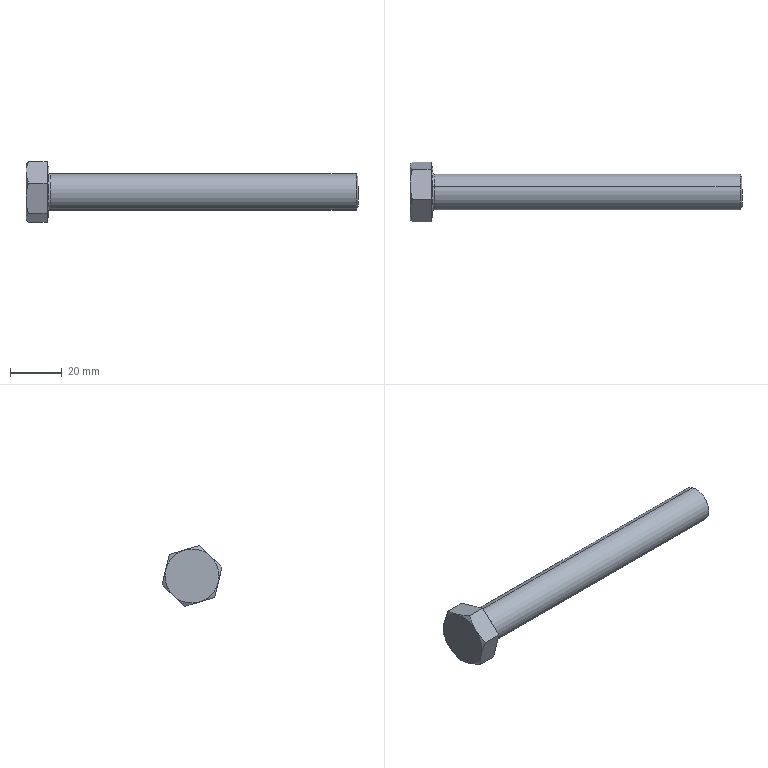Component | SolidWorks | GB_T5785-2016[HexHeadBoltFineThread(M14_1.5)_120]-1 | 1 solid | 24 faces | box 128.8 x 23.23 x 23.59 mm | volume 21766 mm3 | cone 10 | plane 10 | torus 2 | cylinder 2 | commonest cylinder face diameters 14 x2
STEP:
#1=COLOUR_RGB('',0.7922,0.8196,0.9333);
#2=FILL_AREA_STYLE_COLOUR('',#1);
#3=FILL_AREA_STYLE('',(#2));
#4=SURFACE_STYLE_FILL_AREA(#3);
#5=SURFACE_SIDE_STYLE('',(#4));
#6=SURFACE_STYLE_USAGE(.BOTH.,#5);
#7=PRESENTATION_STYLE_ASSIGNMENT((#6));
#8=CARTESIAN_POINT('',(18.543,31.116,10.34));
#9=VERTEX_POINT('',#8);
#10=CARTESIAN_POINT('',(18.543,30.987,9.91));
#11=VERTEX_POINT('',#10);
#12=CARTESIAN_POINT('',(18.543,31.052,10.125));
#13=DIRECTION('',(-1.,-0.,-0.));
#14=DIRECTION('',(-0.,0.2864,0.9581));
#15=AXIS2_PLACEMENT_3D('',#12,#13,#14);
#16=CIRCLE('',#15,0.2244);
#17=EDGE_CURVE('',#9,#11,#16,.T.);
#18=ORIENTED_EDGE('',*,*,#17,.T.);
#19=CARTESIAN_POINT('',(18.513,30.973,9.861));
#20=VERTEX_POINT('',#19);
#21=CARTESIAN_POINT('',(18.513,30.973,9.861));
#22=DIRECTION('',(-0.5,-0.2481,-0.8297));
#23=VECTOR('',#22,39.37);
#24=LINE('',#21,#23);
#25=EDGE_CURVE('',#11,#20,#24,.T.);
#26=ORIENTED_EDGE('',*,*,#25,.T.);
#27=CARTESIAN_POINT('',(18.513,31.13,10.389));
#28=VERTEX_POINT('',#27);
#29=CARTESIAN_POINT('',(18.513,31.052,10.125));
#30=DIRECTION('',(-1.,-0.,-0.));
#31=DIRECTION('',(-0.,0.2864,0.9581));
#32=AXIS2_PLACEMENT_3D('',#29,#30,#31);
#33=CIRCLE('',#32,0.2756);
#34=EDGE_CURVE('',#28,#20,#33,.T.);
#35=ORIENTED_EDGE('',*,*,#34,.F.);
#36=CARTESIAN_POINT('',(18.513,31.13,10.389));
#37=DIRECTION('',(-0.5,0.2481,0.8297));
#38=VECTOR('',#37,39.37);
#39=LINE('',#36,#38);
#40=EDGE_CURVE('',#9,#28,#39,.T.);
#41=ORIENTED_EDGE('',*,*,#40,.F.);
#42=EDGE_LOOP('',(#18,#26,#35,#41));
#43=FACE_OUTER_BOUND('',#42,.T.);
#44=CARTESIAN_POINT('',(18.513,31.052,10.125));
#45=DIRECTION('',(-1.,-0.,-0.));
#46=DIRECTION('',(-0.,0.2864,0.9581));
#47=AXIS2_PLACEMENT_3D('',#44,#45,#46);
#48=CONICAL_SURFACE('',#47,0.2756,1.047);
#49=ADVANCED_FACE('',(#43),#48,.T.);
#50=CARTESIAN_POINT('',(13.842,31.13,10.389));
#51=VERTEX_POINT('',#50);
#52=CARTESIAN_POINT('',(13.842,30.973,9.861));
#53=VERTEX_POINT('',#52);
#54=CARTESIAN_POINT('',(13.842,31.052,10.125));
#55=DIRECTION('',(1.,0.,0.));
#56=DIRECTION('',(0.,-0.2864,-0.9581));
#57=AXIS2_PLACEMENT_3D('',#54,#55,#56);
#58=CIRCLE('',#57,0.2756);
#59=EDGE_CURVE('',#51,#53,#58,.T.);
#60=ORIENTED_EDGE('',*,*,#59,.F.);
#61=CARTESIAN_POINT('',(13.818,31.137,10.412));
#62=VERTEX_POINT('',#61);
#63=CARTESIAN_POINT('',(13.842,31.137,10.412));
#64=DIRECTION('',(-0.,0.9581,-0.2864));
#65=DIRECTION('',(0.,0.2864,0.9581));
#66=AXIS2_PLACEMENT_3D('',#63,#64,#65);
#67=CIRCLE('',#66,0.02362);
#68=EDGE_CURVE('',#51,#62,#67,.T.);
#69=ORIENTED_EDGE('',*,*,#68,.T.);
#70=CARTESIAN_POINT('',(13.818,30.966,9.839));
#71=VERTEX_POINT('',#70);
#72=CARTESIAN_POINT('',(13.818,31.052,10.125));
#73=DIRECTION('',(-1.,-0.,-0.));
#74=DIRECTION('',(0.,-0.2864,-0.9581));
#75=AXIS2_PLACEMENT_3D('',#72,#73,#74);
#76=CIRCLE('',#75,0.2992);
#77=EDGE_CURVE('',#71,#62,#76,.T.);
#78=ORIENTED_EDGE('',*,*,#77,.F.);
#79=CARTESIAN_POINT('',(13.842,30.966,9.839));
#80=DIRECTION('',(0.,-0.9581,0.2864));
#81=DIRECTION('',(0.,-0.2864,-0.9581));
#82=AXIS2_PLACEMENT_3D('',#79,#80,#81);
#83=CIRCLE('',#82,0.02362);
#84=EDGE_CURVE('',#53,#71,#83,.T.);
#85=ORIENTED_EDGE('',*,*,#84,.F.);
#86=EDGE_LOOP('',(#60,#69,#78,#85));
#87=FACE_OUTER_BOUND('',#86,.T.);
#88=CARTESIAN_POINT('',(13.842,31.052,10.125));
#89=DIRECTION('',(1.,0.,0.));
#90=DIRECTION('',(0.,-0.2864,-0.9581));
#91=AXIS2_PLACEMENT_3D('',#88,#89,#90);
#92=TOROIDAL_SURFACE('',#91,0.2992,0.02362);
#93=ADVANCED_FACE('',(#87),#92,.F.);
#94=CARTESIAN_POINT('',(13.818,31.162,10.496));
#95=VERTEX_POINT('',#94);
#96=CARTESIAN_POINT('',(13.818,30.941,9.755));
#97=VERTEX_POINT('',#96);
#98=CARTESIAN_POINT('',(13.818,31.052,10.125));
#99=DIRECTION('',(-1.,-0.,-0.));
#100=DIRECTION('',(-0.,0.2864,0.9581));
#101=AXIS2_PLACEMENT_3D('',#98,#99,#100);
#102=CIRCLE('',#101,0.3866);
#103=EDGE_CURVE('',#95,#97,#102,.T.);
#104=ORIENTED_EDGE('',*,*,#103,.T.);
#105=CARTESIAN_POINT('',(13.795,30.937,9.742));
#106=VERTEX_POINT('',#105);
#107=CARTESIAN_POINT('',(13.795,30.937,9.742));
#108=DIRECTION('',(-0.866,-0.1432,-0.4791));
#109=VECTOR('',#108,39.37);
#110=LINE('',#107,#109);
#111=EDGE_CURVE('',#97,#106,#110,.T.);
#112=ORIENTED_EDGE('',*,*,#111,.T.);
#113=CARTESIAN_POINT('',(13.795,31.166,10.509));
#114=VERTEX_POINT('',#113);
#115=CARTESIAN_POINT('',(13.795,31.052,10.125));
#116=DIRECTION('',(-1.,-0.,-0.));
#117=DIRECTION('',(-0.,0.2864,0.9581));
#118=AXIS2_PLACEMENT_3D('',#115,#116,#117);
#119=CIRCLE('',#118,0.4003);
#120=EDGE_CURVE('',#114,#106,#119,.T.);
#121=ORIENTED_EDGE('',*,*,#120,.F.);
#122=CARTESIAN_POINT('',(13.795,31.166,10.509));
#123=DIRECTION('',(-0.866,0.1432,0.4791));
#124=VECTOR('',#123,39.37);
#125=LINE('',#122,#124);
#126=EDGE_CURVE('',#95,#114,#125,.T.);
#127=ORIENTED_EDGE('',*,*,#126,.F.);
#128=EDGE_LOOP('',(#104,#112,#121,#127));
#129=FACE_OUTER_BOUND('',#128,.T.);
#130=CARTESIAN_POINT('',(13.795,31.052,10.125));
#131=DIRECTION('',(-1.,-0.,-0.));
#132=DIRECTION('',(-0.,0.2864,0.9581));
#133=AXIS2_PLACEMENT_3D('',#130,#131,#132);
#134=CONICAL_SURFACE('',#133,0.4003,0.5236);
#135=ADVANCED_FACE('',(#129),#134,.T.);
#136=ORIENTED_EDGE('',*,*,#34,.T.);
#137=CARTESIAN_POINT('',(13.472,30.973,9.861));
#138=DIRECTION('',(-1.,-0.,-0.));
#139=VECTOR('',#138,39.37);
#140=LINE('',#137,#139);
#141=EDGE_CURVE('',#20,#53,#140,.T.);
#142=ORIENTED_EDGE('',*,*,#141,.T.);
#143=CARTESIAN_POINT('',(13.842,31.052,10.125));
#144=DIRECTION('',(1.,0.,0.));
#145=DIRECTION('',(0.,-0.2864,-0.9581));
#146=AXIS2_PLACEMENT_3D('',#143,#144,#145);
#147=CIRCLE('',#146,0.2756);
#148=EDGE_CURVE('',#53,#51,#147,.T.);
#149=ORIENTED_EDGE('',*,*,#148,.T.);
#150=CARTESIAN_POINT('',(13.472,31.13,10.389));
#151=DIRECTION('',(-1.,-0.,-0.));
#152=VECTOR('',#151,39.37);
#153=LINE('',#150,#152);
#154=EDGE_CURVE('',#28,#51,#153,.T.);
#155=ORIENTED_EDGE('',*,*,#154,.F.);
#156=EDGE_LOOP('',(#136,#142,#149,#155));
#157=FACE_OUTER_BOUND('',#156,.T.);
#158=CARTESIAN_POINT('',(13.472,31.052,10.125));
#159=DIRECTION('',(-1.,-0.,-0.));
#160=DIRECTION('',(-0.,0.2864,0.9581));
#161=AXIS2_PLACEMENT_3D('',#158,#159,#160);
#162=CYLINDRICAL_SURFACE('',#161,0.2756);
#163=ADVANCED_FACE('',(#157),#162,.T.);
#164=ORIENTED_EDGE('',*,*,#141,.F.);
#165=CARTESIAN_POINT('',(18.513,31.052,10.125));
#166=DIRECTION('',(-1.,-0.,-0.));
#167=DIRECTION('',(-0.,0.2864,0.9581));
#168=AXIS2_PLACEMENT_3D('',#165,#166,#167);
#169=CIRCLE('',#168,0.2756);
#170=EDGE_CURVE('',#20,#28,#169,.T.);
#171=ORIENTED_EDGE('',*,*,#170,.T.);
#172=ORIENTED_EDGE('',*,*,#154,.T.);
#173=ORIENTED_EDGE('',*,*,#59,.T.);
#174=EDGE_LOOP('',(#164,#171,#172,#173));
#175=FACE_OUTER_BOUND('',#174,.T.);
#176=CARTESIAN_POINT('',(13.472,31.052,10.125));
#177=DIRECTION('',(-1.,-0.,-0.));
#178=DIRECTION('',(-0.,0.2864,0.9581));
#179=AXIS2_PLACEMENT_3D('',#176,#177,#178);
#180=CYLINDRICAL_SURFACE('',#179,0.2756);
#181=ADVANCED_FACE('',(#175),#180,.T.);
#182=CARTESIAN_POINT('',(13.795,31.162,9.661));
#183=VERTEX_POINT('',#182);
#184=CARTESIAN_POINT('',(13.795,31.509,9.988));
#185=VERTEX_POINT('',#184);
#186=CARTESIAN_POINT('',(13.795,31.162,9.661));
#187=DIRECTION('',(-0.,0.7271,0.6865));
#188=VECTOR('',#187,39.37);
#189=LINE('',#186,#188);
#190=EDGE_CURVE('',#183,#185,#189,.T.);
#191=ORIENTED_EDGE('',*,*,#190,.F.);
#192=CARTESIAN_POINT('',(13.509,31.162,9.661));
#193=VERTEX_POINT('',#192);
#194=CARTESIAN_POINT('',(13.818,31.162,9.661));
#195=DIRECTION('',(-1.,-0.,-0.));
#196=VECTOR('',#195,39.37);
#197=LINE('',#194,#196);
#198=EDGE_CURVE('',#183,#193,#197,.T.);
#199=ORIENTED_EDGE('',*,*,#198,.T.);
#200=CARTESIAN_POINT('',(13.472,31.335,9.825));
#201=VERTEX_POINT('',#200);
#202=CARTESIAN_POINT('',(13.472,31.335,9.825));
#203=CARTESIAN_POINT('',(13.472,31.321,9.811));
#204=CARTESIAN_POINT('',(13.473,31.306,9.797));
#205=CARTESIAN_POINT('',(13.476,31.277,9.769));
#206=CARTESIAN_POINT('',(13.478,31.262,9.755));
#207=CARTESIAN_POINT('',(13.488,31.219,9.714));
#208=CARTESIAN_POINT('',(13.497,31.19,9.687));
#209=CARTESIAN_POINT('',(13.509,31.162,9.661));
#210=B_SPLINE_CURVE_WITH_KNOTS('',3,(#202,#203,#204,#205,#206,#207,#208,#209),.UNSPECIFIED.,.F.,.F.,(4,2,2,4),(0.006134,0.007662,0.00919,0.01225),.UNSPECIFIED.);
#211=EDGE_CURVE('',#201,#193,#210,.T.);
#212=ORIENTED_EDGE('',*,*,#211,.F.);
#213=CARTESIAN_POINT('',(13.509,31.509,9.988));
#214=VERTEX_POINT('',#213);
#215=CARTESIAN_POINT('',(13.509,31.509,9.988));
#216=CARTESIAN_POINT('',(13.497,31.481,9.962));
#217=CARTESIAN_POINT('',(13.488,31.452,9.935));
#218=CARTESIAN_POINT('',(13.475,31.394,9.88));
#219=CARTESIAN_POINT('',(13.472,31.365,9.853));
#220=CARTESIAN_POINT('',(13.472,31.335,9.825));
#221=B_SPLINE_CURVE_WITH_KNOTS('',3,(#215,#216,#217,#218,#219,#220),.UNSPECIFIED.,.F.,.F.,(4,2,4),(0.00000024,0.003067,0.006134),.UNSPECIFIED.);
#222=EDGE_CURVE('',#214,#201,#221,.T.);
#223=ORIENTED_EDGE('',*,*,#222,.F.);
#224=CARTESIAN_POINT('',(13.818,31.509,9.988));
#225=DIRECTION('',(-1.,-0.,-0.));
#226=VECTOR('',#225,39.37);
#227=LINE('',#224,#226);
#228=EDGE_CURVE('',#185,#214,#227,.T.);
#229=ORIENTED_EDGE('',*,*,#228,.F.);
#230=EDGE_LOOP('',(#191,#199,#212,#223,#229));
#231=FACE_OUTER_BOUND('',#230,.T.);
#232=CARTESIAN_POINT('',(13.818,31.162,9.661));
#233=DIRECTION('',(0.,-0.6865,0.7271));
#234=DIRECTION('',(0.,-0.7271,-0.6865));
#235=AXIS2_PLACEMENT_3D('',#232,#233,#234);
#236=PLANE('',#235);
#237=ADVANCED_FACE('',(#231),#236,.F.);
#238=CARTESIAN_POINT('',(13.795,31.399,10.453));
#239=VERTEX_POINT('',#238);
#240=CARTESIAN_POINT('',(13.795,31.509,9.988));
#241=DIRECTION('',(-0.,-0.231,0.973));
#242=VECTOR('',#241,39.37);
#243=LINE('',#240,#242);
#244=EDGE_CURVE('',#185,#239,#243,.T.);
#245=ORIENTED_EDGE('',*,*,#244,.F.);
#246=ORIENTED_EDGE('',*,*,#228,.T.);
#247=CARTESIAN_POINT('',(13.472,31.454,10.221));
#248=VERTEX_POINT('',#247);
#249=CARTESIAN_POINT('',(13.472,31.454,10.221));
#250=CARTESIAN_POINT('',(13.472,31.458,10.201));
#251=CARTESIAN_POINT('',(13.473,31.463,10.181));
#252=CARTESIAN_POINT('',(13.476,31.472,10.142));
#253=CARTESIAN_POINT('',(13.478,31.477,10.123));
#254=CARTESIAN_POINT('',(13.488,31.491,10.065));
#255=CARTESIAN_POINT('',(13.497,31.5,10.026));
#256=CARTESIAN_POINT('',(13.509,31.509,9.988));
#257=B_SPLINE_CURVE_WITH_KNOTS('',3,(#249,#250,#251,#252,#253,#254,#255,#256),.UNSPECIFIED.,.F.,.F.,(4,2,2,4),(0.006134,0.007662,0.00919,0.01225),.UNSPECIFIED.);
#258=EDGE_CURVE('',#248,#214,#257,.T.);
#259=ORIENTED_EDGE('',*,*,#258,.F.);
#260=CARTESIAN_POINT('',(13.509,31.399,10.453));
#261=VERTEX_POINT('',#260);
#262=CARTESIAN_POINT('',(13.509,31.399,10.453));
#263=CARTESIAN_POINT('',(13.497,31.408,10.415));
#264=CARTESIAN_POINT('',(13.488,31.417,10.377));
#265=CARTESIAN_POINT('',(13.475,31.435,10.299));
#266=CARTESIAN_POINT('',(13.472,31.444,10.26));
#267=CARTESIAN_POINT('',(13.472,31.454,10.221));
#268=B_SPLINE_CURVE_WITH_KNOTS('',3,(#262,#263,#264,#265,#266,#267),.UNSPECIFIED.,.F.,.F.,(4,2,4),(0.00000024,0.003067,0.006134),.UNSPECIFIED.);
#269=EDGE_CURVE('',#261,#248,#268,.T.);
#270=ORIENTED_EDGE('',*,*,#269,.F.);
#271=CARTESIAN_POINT('',(13.818,31.399,10.453));
#272=DIRECTION('',(-1.,-0.,-0.));
#273=VECTOR('',#272,39.37);
#274=LINE('',#271,#273);
#275=EDGE_CURVE('',#239,#261,#274,.T.);
#276=ORIENTED_EDGE('',*,*,#275,.F.);
#277=EDGE_LOOP('',(#245,#246,#259,#270,#276));
#278=FACE_OUTER_BOUND('',#277,.T.);
#279=CARTESIAN_POINT('',(13.818,31.509,9.988));
#280=DIRECTION('',(0.,-0.973,-0.231));
#281=DIRECTION('',(0.,0.231,-0.973));
#282=AXIS2_PLACEMENT_3D('',#279,#280,#281);
#283=PLANE('',#282);
#284=ADVANCED_FACE('',(#278),#283,.F.);
#285=CARTESIAN_POINT('',(13.795,30.941,10.59));
#286=VERTEX_POINT('',#285);
#287=CARTESIAN_POINT('',(13.795,31.399,10.453));
#288=DIRECTION('',(0.,-0.9581,0.2864));
#289=VECTOR('',#288,39.37);
#290=LINE('',#287,#289);
#291=EDGE_CURVE('',#239,#286,#290,.T.);
#292=ORIENTED_EDGE('',*,*,#291,.F.);
#293=ORIENTED_EDGE('',*,*,#275,.T.);
#294=CARTESIAN_POINT('',(13.472,31.17,10.521));
#295=VERTEX_POINT('',#294);
#296=CARTESIAN_POINT('',(13.472,31.17,10.521));
#297=CARTESIAN_POINT('',(13.472,31.189,10.515));
#298=CARTESIAN_POINT('',(13.473,31.209,10.51));
#299=CARTESIAN_POINT('',(13.476,31.248,10.498));
#300=CARTESIAN_POINT('',(13.478,31.267,10.492));
#301=CARTESIAN_POINT('',(13.488,31.324,10.475));
#302=CARTESIAN_POINT('',(13.497,31.362,10.464));
#303=CARTESIAN_POINT('',(13.509,31.399,10.453));
#304=B_SPLINE_CURVE_WITH_KNOTS('',3,(#296,#297,#298,#299,#300,#301,#302,#303),.UNSPECIFIED.,.F.,.F.,(4,2,2,4),(0.0174,0.01894,0.02047,0.02354),.UNSPECIFIED.);
#305=EDGE_CURVE('',#295,#261,#304,.T.);
#306=ORIENTED_EDGE('',*,*,#305,.F.);
#307=CARTESIAN_POINT('',(13.509,30.941,10.59));
#308=VERTEX_POINT('',#307);
#309=CARTESIAN_POINT('',(13.509,30.941,10.59));
#310=CARTESIAN_POINT('',(13.497,30.979,10.578));
#311=CARTESIAN_POINT('',(13.488,31.017,10.567));
#312=CARTESIAN_POINT('',(13.475,31.093,10.544));
#313=CARTESIAN_POINT('',(13.472,31.131,10.533));
#314=CARTESIAN_POINT('',(13.472,31.17,10.521));
#315=B_SPLINE_CURVE_WITH_KNOTS('',3,(#309,#310,#311,#312,#313,#314),.UNSPECIFIED.,.F.,.F.,(4,2,4),(0.01126,0.01433,0.0174),.UNSPECIFIED.);
#316=EDGE_CURVE('',#308,#295,#315,.T.);
#317=ORIENTED_EDGE('',*,*,#316,.F.);
#318=CARTESIAN_POINT('',(13.818,30.941,10.59));
#319=DIRECTION('',(-1.,-0.,-0.));
#320=VECTOR('',#319,39.37);
#321=LINE('',#318,#320);
#322=EDGE_CURVE('',#286,#308,#321,.T.);
#323=ORIENTED_EDGE('',*,*,#322,.F.);
#324=EDGE_LOOP('',(#292,#293,#306,#317,#323));
#325=FACE_OUTER_BOUND('',#324,.T.);
#326=CARTESIAN_POINT('',(13.818,31.399,10.453));
#327=DIRECTION('',(0.,-0.2864,-0.9581));
#328=DIRECTION('',(-0.,0.9581,-0.2864));
#329=AXIS2_PLACEMENT_3D('',#326,#327,#328);
#330=PLANE('',#329);
#331=ADVANCED_FACE('',(#325),#330,.F.);
#332=CARTESIAN_POINT('',(13.795,30.594,10.262));
#333=VERTEX_POINT('',#332);
#334=CARTESIAN_POINT('',(13.795,30.594,10.262));
#335=DIRECTION('',(0.,-0.7271,-0.6865));
#336=VECTOR('',#335,39.37);
#337=LINE('',#334,#336);
#338=EDGE_CURVE('',#286,#333,#337,.T.);
#339=ORIENTED_EDGE('',*,*,#338,.F.);
#340=ORIENTED_EDGE('',*,*,#322,.T.);
#341=CARTESIAN_POINT('',(13.472,30.768,10.426));
#342=VERTEX_POINT('',#341);
#343=CARTESIAN_POINT('',(13.472,30.768,10.426));
#344=CARTESIAN_POINT('',(13.472,30.782,10.44));
#345=CARTESIAN_POINT('',(13.473,30.797,10.454));
#346=CARTESIAN_POINT('',(13.476,30.827,10.481));
#347=CARTESIAN_POINT('',(13.478,30.841,10.495));
#348=CARTESIAN_POINT('',(13.488,30.884,10.536));
#349=CARTESIAN_POINT('',(13.497,30.913,10.563));
#350=CARTESIAN_POINT('',(13.509,30.941,10.59));
#351=B_SPLINE_CURVE_WITH_KNOTS('',3,(#343,#344,#345,#346,#347,#348,#349,#350),.UNSPECIFIED.,.F.,.F.,(4,2,2,4),(0.006134,0.007662,0.00919,0.01225),.UNSPECIFIED.);
#352=EDGE_CURVE('',#342,#308,#351,.T.);
#353=ORIENTED_EDGE('',*,*,#352,.F.);
#354=CARTESIAN_POINT('',(13.509,30.594,10.262));
#355=VERTEX_POINT('',#354);
#356=CARTESIAN_POINT('',(13.509,30.594,10.262));
#357=CARTESIAN_POINT('',(13.497,30.623,10.289));
#358=CARTESIAN_POINT('',(13.488,30.651,10.316));
#359=CARTESIAN_POINT('',(13.475,30.709,10.37));
#360=CARTESIAN_POINT('',(13.472,30.738,10.398));
#361=CARTESIAN_POINT('',(13.472,30.768,10.426));
#362=B_SPLINE_CURVE_WITH_KNOTS('',3,(#356,#357,#358,#359,#360,#361),.UNSPECIFIED.,.F.,.F.,(4,2,4),(0.00000024,0.003067,0.006134),.UNSPECIFIED.);
#363=EDGE_CURVE('',#355,#342,#362,.T.);
#364=ORIENTED_EDGE('',*,*,#363,.F.);
#365=CARTESIAN_POINT('',(13.818,30.594,10.262));
#366=DIRECTION('',(-1.,-0.,-0.));
#367=VECTOR('',#366,39.37);
#368=LINE('',#365,#367);
#369=EDGE_CURVE('',#333,#355,#368,.T.);
#370=ORIENTED_EDGE('',*,*,#369,.F.);
#371=EDGE_LOOP('',(#339,#340,#353,#364,#370));
#372=FACE_OUTER_BOUND('',#371,.T.);
#373=CARTESIAN_POINT('',(13.818,30.594,10.262));
#374=DIRECTION('',(-0.,0.6865,-0.7271));
#375=DIRECTION('',(-0.,0.7271,0.6865));
#376=AXIS2_PLACEMENT_3D('',#373,#374,#375);
#377=PLANE('',#376);
#378=ADVANCED_FACE('',(#372),#377,.F.);
#379=CARTESIAN_POINT('',(13.795,30.704,9.797));
#380=VERTEX_POINT('',#379);
#381=CARTESIAN_POINT('',(13.795,30.704,9.797));
#382=DIRECTION('',(0.,0.231,-0.973));
#383=VECTOR('',#382,39.37);
#384=LINE('',#381,#383);
#385=EDGE_CURVE('',#333,#380,#384,.T.);
#386=ORIENTED_EDGE('',*,*,#385,.F.);
#387=ORIENTED_EDGE('',*,*,#369,.T.);
#388=CARTESIAN_POINT('',(13.472,30.649,10.03));
#389=VERTEX_POINT('',#388);
#390=CARTESIAN_POINT('',(13.472,30.649,10.03));
#391=CARTESIAN_POINT('',(13.472,30.645,10.049));
#392=CARTESIAN_POINT('',(13.473,30.64,10.069));
#393=CARTESIAN_POINT('',(13.476,30.631,10.108));
#394=CARTESIAN_POINT('',(13.478,30.626,10.128));
#395=CARTESIAN_POINT('',(13.488,30.612,10.186));
#396=CARTESIAN_POINT('',(13.497,30.603,10.224));
#397=CARTESIAN_POINT('',(13.509,30.594,10.262));
#398=B_SPLINE_CURVE_WITH_KNOTS('',3,(#390,#391,#392,#393,#394,#395,#396,#397),.UNSPECIFIED.,.F.,.F.,(4,2,2,4),(0.006134,0.007662,0.00919,0.01225),.UNSPECIFIED.);
#399=EDGE_CURVE('',#389,#355,#398,.T.);
#400=ORIENTED_EDGE('',*,*,#399,.F.);
#401=CARTESIAN_POINT('',(13.509,30.704,9.797));
#402=VERTEX_POINT('',#401);
#403=CARTESIAN_POINT('',(13.509,30.704,9.797));
#404=CARTESIAN_POINT('',(13.497,30.695,9.835));
#405=CARTESIAN_POINT('',(13.488,30.686,9.874));
#406=CARTESIAN_POINT('',(13.475,30.668,9.951));
#407=CARTESIAN_POINT('',(13.472,30.659,9.99));
#408=CARTESIAN_POINT('',(13.472,30.649,10.03));
#409=B_SPLINE_CURVE_WITH_KNOTS('',3,(#403,#404,#405,#406,#407,#408),.UNSPECIFIED.,.F.,.F.,(4,2,4),(0.00000024,0.003067,0.006134),.UNSPECIFIED.);
#410=EDGE_CURVE('',#402,#389,#409,.T.);
#411=ORIENTED_EDGE('',*,*,#410,.F.);
#412=CARTESIAN_POINT('',(13.818,30.704,9.797));
#413=DIRECTION('',(-1.,-0.,-0.));
#414=VECTOR('',#413,39.37);
#415=LINE('',#412,#414);
#416=EDGE_CURVE('',#380,#402,#415,.T.);
#417=ORIENTED_EDGE('',*,*,#416,.F.);
#418=EDGE_LOOP('',(#386,#387,#400,#411,#417));
#419=FACE_OUTER_BOUND('',#418,.T.);
#420=CARTESIAN_POINT('',(13.818,30.704,9.797));
#421=DIRECTION('',(-0.,0.973,0.231));
#422=DIRECTION('',(-0.,-0.231,0.973));
#423=AXIS2_PLACEMENT_3D('',#420,#421,#422);
#424=PLANE('',#423);
#425=ADVANCED_FACE('',(#419),#424,.F.);
#426=CARTESIAN_POINT('',(13.795,31.162,9.661));
#427=DIRECTION('',(-0.,0.9581,-0.2864));
#428=VECTOR('',#427,39.37);
#429=LINE('',#426,#428);
#430=EDGE_CURVE('',#380,#183,#429,.T.);
#431=ORIENTED_EDGE('',*,*,#430,.F.);
#432=ORIENTED_EDGE('',*,*,#416,.T.);
#433=CARTESIAN_POINT('',(13.472,30.933,9.729));
#434=VERTEX_POINT('',#433);
#435=CARTESIAN_POINT('',(13.472,30.933,9.729));
#436=CARTESIAN_POINT('',(13.472,30.894,9.741));
#437=CARTESIAN_POINT('',(13.475,30.856,9.752));
#438=CARTESIAN_POINT('',(13.488,30.78,9.775));
#439=CARTESIAN_POINT('',(13.497,30.742,9.786));
#440=CARTESIAN_POINT('',(13.509,30.704,9.797));
#441=B_SPLINE_CURVE_WITH_KNOTS('',3,(#435,#436,#437,#438,#439,#440),.UNSPECIFIED.,.F.,.F.,(4,2,4),(0.03489,0.03796,0.04103),.UNSPECIFIED.);
#442=EDGE_CURVE('',#434,#402,#441,.T.);
#443=ORIENTED_EDGE('',*,*,#442,.F.);
#444=CARTESIAN_POINT('',(13.509,31.162,9.661));
#445=CARTESIAN_POINT('',(13.497,31.125,9.672));
#446=CARTESIAN_POINT('',(13.488,31.087,9.683));
#447=CARTESIAN_POINT('',(13.478,31.03,9.7));
#448=CARTESIAN_POINT('',(13.476,31.011,9.706));
#449=CARTESIAN_POINT('',(13.473,30.972,9.717));
#450=CARTESIAN_POINT('',(13.472,30.953,9.723));
#451=CARTESIAN_POINT('',(13.472,30.933,9.729));
#452=B_SPLINE_CURVE_WITH_KNOTS('',3,(#444,#445,#446,#447,#448,#449,#450,#451),.UNSPECIFIED.,.F.,.F.,(4,2,2,4),(0.02875,0.03182,0.03336,0.03489),.UNSPECIFIED.);
#453=EDGE_CURVE('',#193,#434,#452,.T.);
#454=ORIENTED_EDGE('',*,*,#453,.F.);
#455=ORIENTED_EDGE('',*,*,#198,.F.);
#456=EDGE_LOOP('',(#431,#432,#443,#454,#455));
#457=FACE_OUTER_BOUND('',#456,.T.);
#458=CARTESIAN_POINT('',(13.818,31.162,9.661));
#459=DIRECTION('',(-0.,0.2864,0.9581));
#460=DIRECTION('',(0.,-0.9581,0.2864));
#461=AXIS2_PLACEMENT_3D('',#458,#459,#460);
#462=PLANE('',#461);
#463=ADVANCED_FACE('',(#457),#462,.F.);
#464=ORIENTED_EDGE('',*,*,#410,.T.);
#465=CARTESIAN_POINT('',(13.472,31.052,10.125));
#466=DIRECTION('',(1.,0.,0.));
#467=DIRECTION('',(0.,-0.2864,-0.9581));
#468=AXIS2_PLACEMENT_3D('',#465,#466,#467);
#469=CIRCLE('',#468,0.4134);
#470=EDGE_CURVE('',#389,#434,#469,.T.);
#471=ORIENTED_EDGE('',*,*,#470,.T.);
#472=ORIENTED_EDGE('',*,*,#442,.T.);
#473=EDGE_LOOP('',(#464,#471,#472));
#474=FACE_OUTER_BOUND('',#473,.T.);
#475=CARTESIAN_POINT('',(13.472,31.052,10.125));
#476=DIRECTION('',(1.,0.,0.));
#477=DIRECTION('',(0.,-0.2864,-0.9581));
#478=AXIS2_PLACEMENT_3D('',#475,#476,#477);
#479=CONICAL_SURFACE('',#478,0.4134,1.047);
#480=ADVANCED_FACE('',(#474),#479,.T.);
#481=ORIENTED_EDGE('',*,*,#363,.T.);
#482=CARTESIAN_POINT('',(13.472,31.052,10.125));
#483=DIRECTION('',(1.,0.,0.));
#484=DIRECTION('',(0.,-0.2864,-0.9581));
#485=AXIS2_PLACEMENT_3D('',#482,#483,#484);
#486=CIRCLE('',#485,0.4134);
#487=EDGE_CURVE('',#342,#389,#486,.T.);
#488=ORIENTED_EDGE('',*,*,#487,.T.);
#489=ORIENTED_EDGE('',*,*,#399,.T.);
#490=EDGE_LOOP('',(#481,#488,#489));
#491=FACE_OUTER_BOUND('',#490,.T.);
#492=CARTESIAN_POINT('',(13.472,31.052,10.125));
#493=DIRECTION('',(1.,0.,0.));
#494=DIRECTION('',(0.,-0.2864,-0.9581));
#495=AXIS2_PLACEMENT_3D('',#492,#493,#494);
#496=CONICAL_SURFACE('',#495,0.4134,1.047);
#497=ADVANCED_FACE('',(#491),#496,.T.);
#498=ORIENTED_EDGE('',*,*,#316,.T.);
#499=CARTESIAN_POINT('',(13.472,31.052,10.125));
#500=DIRECTION('',(1.,0.,0.));
#501=DIRECTION('',(0.,-0.2864,-0.9581));
#502=AXIS2_PLACEMENT_3D('',#499,#500,#501);
#503=CIRCLE('',#502,0.4134);
#504=EDGE_CURVE('',#295,#342,#503,.T.);
#505=ORIENTED_EDGE('',*,*,#504,.T.);
#506=ORIENTED_EDGE('',*,*,#352,.T.);
#507=EDGE_LOOP('',(#498,#505,#506));
#508=FACE_OUTER_BOUND('',#507,.T.);
#509=CARTESIAN_POINT('',(13.472,31.052,10.125));
#510=DIRECTION('',(1.,0.,0.));
#511=DIRECTION('',(0.,-0.2864,-0.9581));
#512=AXIS2_PLACEMENT_3D('',#509,#510,#511);
#513=CONICAL_SURFACE('',#512,0.4134,1.047);
#514=ADVANCED_FACE('',(#508),#513,.T.);
#515=ORIENTED_EDGE('',*,*,#305,.T.);
#516=ORIENTED_EDGE('',*,*,#269,.T.);
#517=CARTESIAN_POINT('',(13.472,31.052,10.125));
#518=DIRECTION('',(-1.,-0.,-0.));
#519=DIRECTION('',(-0.,0.2864,0.9581));
#520=AXIS2_PLACEMENT_3D('',#517,#518,#519);
#521=CIRCLE('',#520,0.4134);
#522=EDGE_CURVE('',#295,#248,#521,.T.);
#523=ORIENTED_EDGE('',*,*,#522,.F.);
#524=EDGE_LOOP('',(#515,#516,#523));
#525=FACE_OUTER_BOUND('',#524,.T.);
#526=CARTESIAN_POINT('',(13.472,31.052,10.125));
#527=DIRECTION('',(1.,0.,0.));
#528=DIRECTION('',(0.,-0.2864,-0.9581));
#529=AXIS2_PLACEMENT_3D('',#526,#527,#528);
#530=CONICAL_SURFACE('',#529,0.4134,1.047);
#531=ADVANCED_FACE('',(#525),#530,.T.);
#532=ORIENTED_EDGE('',*,*,#258,.T.);
#533=ORIENTED_EDGE('',*,*,#222,.T.);
#534=CARTESIAN_POINT('',(13.472,31.052,10.125));
#535=DIRECTION('',(1.,0.,0.));
#536=DIRECTION('',(0.,-0.2864,-0.9581));
#537=AXIS2_PLACEMENT_3D('',#534,#535,#536);
#538=CIRCLE('',#537,0.4134);
#539=EDGE_CURVE('',#201,#248,#538,.T.);
#540=ORIENTED_EDGE('',*,*,#539,.T.);
#541=EDGE_LOOP('',(#532,#533,#540));
#542=FACE_OUTER_BOUND('',#541,.T.);
#543=CARTESIAN_POINT('',(13.472,31.052,10.125));
#544=DIRECTION('',(1.,0.,0.));
#545=DIRECTION('',(0.,-0.2864,-0.9581));
#546=AXIS2_PLACEMENT_3D('',#543,#544,#545);
#547=CONICAL_SURFACE('',#546,0.4134,1.047);
#548=ADVANCED_FACE('',(#542),#547,.T.);
#549=ORIENTED_EDGE('',*,*,#211,.T.);
#550=ORIENTED_EDGE('',*,*,#453,.T.);
#551=CARTESIAN_POINT('',(13.472,31.052,10.125));
#552=DIRECTION('',(1.,0.,0.));
#553=DIRECTION('',(0.,-0.2864,-0.9581));
#554=AXIS2_PLACEMENT_3D('',#551,#552,#553);
#555=CIRCLE('',#554,0.4134);
#556=EDGE_CURVE('',#434,#201,#555,.T.);
#557=ORIENTED_EDGE('',*,*,#556,.T.);
#558=EDGE_LOOP('',(#549,#550,#557));
#559=FACE_OUTER_BOUND('',#558,.T.);
#560=CARTESIAN_POINT('',(13.472,31.052,10.125));
#561=DIRECTION('',(1.,0.,0.));
#562=DIRECTION('',(0.,-0.2864,-0.9581));
#563=AXIS2_PLACEMENT_3D('',#560,#561,#562);
#564=CONICAL_SURFACE('',#563,0.4134,1.047);
#565=ADVANCED_FACE('',(#559),#564,.T.);
#566=ORIENTED_EDGE('',*,*,#556,.F.);
#567=ORIENTED_EDGE('',*,*,#470,.F.);
#568=ORIENTED_EDGE('',*,*,#487,.F.);
#569=ORIENTED_EDGE('',*,*,#504,.F.);
#570=ORIENTED_EDGE('',*,*,#522,.T.);
#571=ORIENTED_EDGE('',*,*,#539,.F.);
#572=EDGE_LOOP('',(#566,#567,#568,#569,#570,#571));
#573=FACE_OUTER_BOUND('',#572,.T.);
#574=CARTESIAN_POINT('',(13.472,31.509,9.988));
#575=DIRECTION('',(1.,0.,0.));
#576=DIRECTION('',(0.,-0.2864,-0.9581));
#577=AXIS2_PLACEMENT_3D('',#574,#575,#576);
#578=PLANE('',#577);
#579=ADVANCED_FACE('',(#573),#578,.F.);
#580=ORIENTED_EDGE('',*,*,#120,.T.);
#581=CARTESIAN_POINT('',(13.795,31.052,10.125));
#582=DIRECTION('',(-1.,-0.,-0.));
#583=DIRECTION('',(-0.,0.2864,0.9581));
#584=AXIS2_PLACEMENT_3D('',#581,#582,#583);
#585=CIRCLE('',#584,0.4003);
#586=EDGE_CURVE('',#106,#114,#585,.T.);
#587=ORIENTED_EDGE('',*,*,#586,.T.);
#588=EDGE_LOOP('',(#580,#587));
#589=FACE_BOUND('',#588,.T.);
#590=ORIENTED_EDGE('',*,*,#190,.T.);
#591=ORIENTED_EDGE('',*,*,#244,.T.);
#592=ORIENTED_EDGE('',*,*,#291,.T.);
#593=ORIENTED_EDGE('',*,*,#338,.T.);
#594=ORIENTED_EDGE('',*,*,#385,.T.);
#595=ORIENTED_EDGE('',*,*,#430,.T.);
#596=EDGE_LOOP('',(#590,#591,#592,#593,#594,#595));
#597=FACE_OUTER_BOUND('',#596,.T.);
#598=CARTESIAN_POINT('',(13.795,31.435,10.011));
#599=DIRECTION('',(1.,0.,0.));
#600=DIRECTION('',(0.,-0.2864,-0.9581));
#601=AXIS2_PLACEMENT_3D('',#598,#599,#600);
#602=PLANE('',#601);
#603=ADVANCED_FACE('',(#589,#597),#602,.T.);
#604=ORIENTED_EDGE('',*,*,#111,.F.);
#605=CARTESIAN_POINT('',(13.818,31.052,10.125));
#606=DIRECTION('',(-1.,-0.,-0.));
#607=DIRECTION('',(-0.,0.2864,0.9581));
#608=AXIS2_PLACEMENT_3D('',#605,#606,#607);
#609=CIRCLE('',#608,0.3866);
#610=EDGE_CURVE('',#97,#95,#609,.T.);
#611=ORIENTED_EDGE('',*,*,#610,.T.);
#612=ORIENTED_EDGE('',*,*,#126,.T.);
#613=ORIENTED_EDGE('',*,*,#586,.F.);
#614=EDGE_LOOP('',(#604,#611,#612,#613));
#615=FACE_OUTER_BOUND('',#614,.T.);
#616=CARTESIAN_POINT('',(13.795,31.052,10.125));
#617=DIRECTION('',(-1.,-0.,-0.));
#618=DIRECTION('',(-0.,0.2864,0.9581));
#619=AXIS2_PLACEMENT_3D('',#616,#617,#618);
#620=CONICAL_SURFACE('',#619,0.4003,0.5236);
#621=ADVANCED_FACE('',(#615),#620,.T.);
#622=ORIENTED_EDGE('',*,*,#77,.T.);
#623=CARTESIAN_POINT('',(13.818,31.052,10.125));
#624=DIRECTION('',(-1.,-0.,-0.));
#625=DIRECTION('',(0.,-0.2864,-0.9581));
#626=AXIS2_PLACEMENT_3D('',#623,#624,#625);
#627=CIRCLE('',#626,0.2992);
#628=EDGE_CURVE('',#62,#71,#627,.T.);
#629=ORIENTED_EDGE('',*,*,#628,.T.);
#630=EDGE_LOOP('',(#622,#629));
#631=FACE_BOUND('',#630,.T.);
#632=ORIENTED_EDGE('',*,*,#103,.F.);
#633=ORIENTED_EDGE('',*,*,#610,.F.);
#634=EDGE_LOOP('',(#632,#633));
#635=FACE_OUTER_BOUND('',#634,.T.);
#636=CARTESIAN_POINT('',(13.818,31.509,9.988));
#637=DIRECTION('',(1.,0.,0.));
#638=DIRECTION('',(0.,-0.2864,-0.9581));
#639=AXIS2_PLACEMENT_3D('',#636,#637,#638);
#640=PLANE('',#639);
#641=ADVANCED_FACE('',(#631,#635),#640,.T.);
#642=ORIENTED_EDGE('',*,*,#68,.F.);
#643=ORIENTED_EDGE('',*,*,#148,.F.);
#644=ORIENTED_EDGE('',*,*,#84,.T.);
#645=ORIENTED_EDGE('',*,*,#628,.F.);
#646=EDGE_LOOP('',(#642,#643,#644,#645));
#647=FACE_OUTER_BOUND('',#646,.T.);
#648=CARTESIAN_POINT('',(13.842,31.052,10.125));
#649=DIRECTION('',(1.,0.,0.));
#650=DIRECTION('',(0.,-0.2864,-0.9581));
#651=AXIS2_PLACEMENT_3D('',#648,#649,#650);
#652=TOROIDAL_SURFACE('',#651,0.2992,0.02362);
#653=ADVANCED_FACE('',(#647),#652,.F.);
#654=ORIENTED_EDGE('',*,*,#25,.F.);
#655=CARTESIAN_POINT('',(18.543,31.052,10.125));
#656=DIRECTION('',(-1.,-0.,-0.));
#657=DIRECTION('',(-0.,0.2864,0.9581));
#658=AXIS2_PLACEMENT_3D('',#655,#656,#657);
#659=CIRCLE('',#658,0.2244);
#660=EDGE_CURVE('',#11,#9,#659,.T.);
#661=ORIENTED_EDGE('',*,*,#660,.T.);
#662=ORIENTED_EDGE('',*,*,#40,.T.);
#663=ORIENTED_EDGE('',*,*,#170,.F.);
#664=EDGE_LOOP('',(#654,#661,#662,#663));
#665=FACE_OUTER_BOUND('',#664,.T.);
#666=CARTESIAN_POINT('',(18.513,31.052,10.125));
#667=DIRECTION('',(-1.,-0.,-0.));
#668=DIRECTION('',(-0.,0.2864,0.9581));
#669=AXIS2_PLACEMENT_3D('',#666,#667,#668);
#670=CONICAL_SURFACE('',#669,0.2756,1.047);
#671=ADVANCED_FACE('',(#665),#670,.T.);
#672=ORIENTED_EDGE('',*,*,#17,.F.);
#673=ORIENTED_EDGE('',*,*,#660,.F.);
#674=EDGE_LOOP('',(#672,#673));
#675=FACE_OUTER_BOUND('',#674,.T.);
#676=CARTESIAN_POINT('',(18.543,31.052,10.125));
#677=DIRECTION('',(-1.,-0.,-0.));
#678=DIRECTION('',(-0.,0.2864,0.9581));
#679=AXIS2_PLACEMENT_3D('',#676,#677,#678);
#680=PLANE('',#679);
#681=ADVANCED_FACE('',(#675),#680,.F.);
#682=CLOSED_SHELL('',(#49,#93,#135,#163,#181,#237,#284,#331,#378,#425,#463,#480,#497,#514,#531,#548,#565,#579,#603,#621,#641,#653,#671,#681));
#683=MANIFOLD_SOLID_BREP('',#682);
#684=STYLED_ITEM('',(#7),#683);
#685=(LENGTH_UNIT()NAMED_UNIT(*)SI_UNIT($,.METRE.));
#686=LENGTH_MEASURE_WITH_UNIT(LENGTH_MEASURE(0.0254),#685);
#687=DIMENSIONAL_EXPONENTS(1.,0.,0.,0.,0.,0.,0.);
#688=(CONVERSION_BASED_UNIT('',#686)LENGTH_UNIT()NAMED_UNIT(#687));
#689=UNCERTAINTY_MEASURE_WITH_UNIT(LENGTH_MEASURE(0.00001),#688,'','');
#690=(NAMED_UNIT(*)PLANE_ANGLE_UNIT()SI_UNIT($,.RADIAN.));
#691=(NAMED_UNIT(*)SI_UNIT($,.STERADIAN.)SOLID_ANGLE_UNIT());
#692=(GEOMETRIC_REPRESENTATION_CONTEXT(3)GLOBAL_UNCERTAINTY_ASSIGNED_CONTEXT((#689))GLOBAL_UNIT_ASSIGNED_CONTEXT((#688,#690,#691))REPRESENTATION_CONTEXT('',''));
#693=MECHANICAL_DESIGN_GEOMETRIC_PRESENTATION_REPRESENTATION('',(#684),#692);
#694=PRESENTATION_LAYER_ASSIGNMENT('','',(#684));
#695=CARTESIAN_POINT('',(0.,0.,0.));
#696=DIRECTION('',(0.,0.,1.));
#697=DIRECTION('',(1.,0.,0.));
#698=AXIS2_PLACEMENT_3D('',#695,#696,#697);
#699=(LENGTH_UNIT()NAMED_UNIT(*)SI_UNIT($,.METRE.));
#700=LENGTH_MEASURE_WITH_UNIT(LENGTH_MEASURE(0.0254),#699);
#701=DIMENSIONAL_EXPONENTS(1.,0.,0.,0.,0.,0.,0.);
#702=(CONVERSION_BASED_UNIT('',#700)LENGTH_UNIT()NAMED_UNIT(#701));
#703=UNCERTAINTY_MEASURE_WITH_UNIT(LENGTH_MEASURE(0.00001),#702,'','');
#704=(NAMED_UNIT(*)PLANE_ANGLE_UNIT()SI_UNIT($,.RADIAN.));
#705=(NAMED_UNIT(*)SI_UNIT($,.STERADIAN.)SOLID_ANGLE_UNIT());
#706=(GEOMETRIC_REPRESENTATION_CONTEXT(3)GLOBAL_UNCERTAINTY_ASSIGNED_CONTEXT((#703))GLOBAL_UNIT_ASSIGNED_CONTEXT((#702,#704,#705))REPRESENTATION_CONTEXT('',''));
#707=ADVANCED_BREP_SHAPE_REPRESENTATION('',(#683,#698),#706);